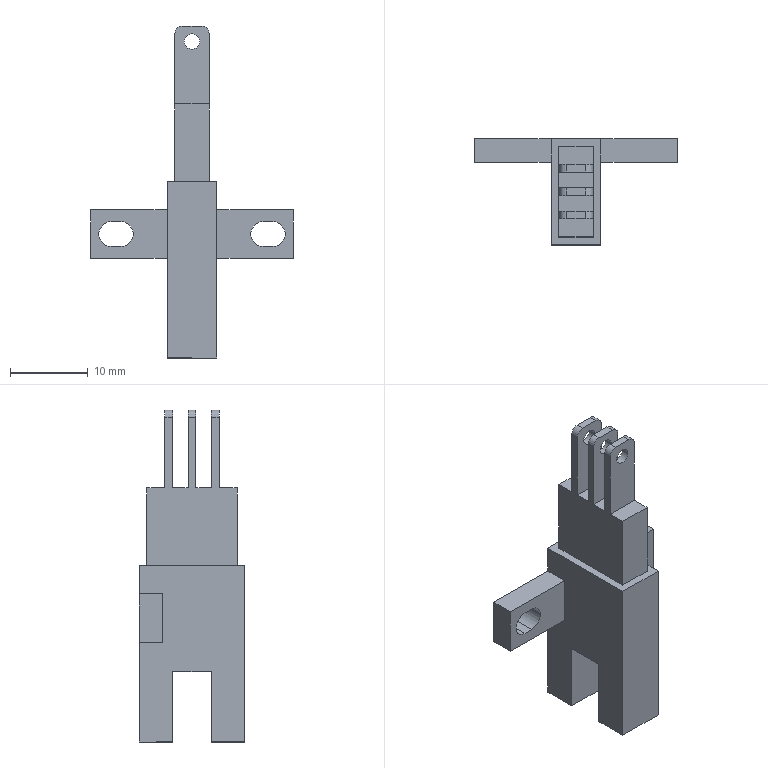Component | SolidWorks | U-shapedSensor-1 | 1 solid | 55 faces | box 26 x 13.6 x 42.6 mm | volume 2610 mm3 | plane 39 | cylinder 16 | commonest cylinder face diameters 2 x12 3.2 x4
build123d program:
from build123d import *

# Parameters (mm, degrees)
SKETCH1_W              = 13.6
SKETCH1_H              = 22.6
BOSS_EXTRUDE1_DEPTH    = 6.4
SKETCH2_W              = 4.9
SKETCH2_H              = 9
CUT_EXTRUDE1_DEPTH     = 28.142
SKETCH3_W              = 13
SKETCH3_H              = 6.2
BOSS_EXTRUDE2_DEPTH    = 3
CUT_EXTRUDE2_DEPTH     = 31.954
SKETCH5_W              = 11.6
SKETCH5_H              = 4.4
BOSS_EXTRUDE3_DEPTH    = 10
SKETCH6_W              = 1
SKETCH6_H              = 4.4
BOSS_EXTRUDE4_DEPTH    = 10
FILLET1_R              = 1
SKETCH7_R              = 1
CUT_EXTRUDE3_DEPTH     = 10
LPATTERN1_COUNT        = 2
LPATTERN1_PITCH        = 3
LPATTERN1_COUNT_DIR2   = 2
LPATTERN1_PITCH_DIR2   = 3
FILLET1_OF_LPATTERN1_R = 1


with BuildPart() as part:
    # Sketch1 → Boss-Extrude1 (new body)
    with BuildSketch(Plane.XY):
        with Locations((6.8, -11.3)):
            Rectangle(SKETCH1_W, SKETCH1_H)
    extrude(amount=BOSS_EXTRUDE1_DEPTH)

    # Sketch2 → Cut-Extrude1 (cut, through all)
    with BuildSketch(Plane.XY.offset(6.4)):
        with Locations((6.8, -4.5)):
            Rectangle(SKETCH2_W, SKETCH2_H)
    extrude(amount=-CUT_EXTRUDE1_DEPTH, mode=Mode.SUBTRACT)

    # Sketch3 → Boss-Extrude2 (add)
    with BuildSketch(Plane.ZY):
        with Locations((9.7, -15.9)):
            Rectangle(SKETCH3_W, SKETCH3_H)
    boss_extrude2 = extrude(amount=-BOSS_EXTRUDE2_DEPTH)

    # Sketch4 → Cut-Extrude2 (cut, through all)
    with BuildSketch(Plane.ZY):
        with BuildLine():
            Line((12.35, -14.3), (13.55, -14.3))
            ThreePointArc((13.55, -14.3), (15.15, -15.9), (13.55, -17.5))
            Line((13.55, -17.5), (12.35, -17.5))
            ThreePointArc((12.35, -17.5), (10.75, -15.9), (12.35, -14.3))
        make_face()
    cut_extrude2 = extrude(amount=-CUT_EXTRUDE2_DEPTH, mode=Mode.SUBTRACT)

    # Mirror1: Boss-Extrude2, Cut-Extrude2 across plane
    add(boss_extrude2.mirror(Plane(origin=(0, 0, 3.2), x_dir=(1, 0, 0), z_dir=(0, 0, -1))))
    add(cut_extrude2.mirror(Plane(origin=(0, 0, 3.2), x_dir=(1, 0, 0), z_dir=(0, 0, -1))), mode=Mode.SUBTRACT)

    # Sketch5 → Boss-Extrude3 (add)
    with BuildSketch(Plane.XZ.offset(22.6)):
        with Locations((6.8, 3.2)):
            Rectangle(SKETCH5_W, SKETCH5_H)
    extrude(amount=BOSS_EXTRUDE3_DEPTH)

    # Sketch6 → Boss-Extrude4 (add)
    with BuildSketch(Plane.XZ.offset(32.6)):
        with Locations((6.8, 3.2)):
            Rectangle(SKETCH6_W, SKETCH6_H)
    boss_extrude4 = extrude(amount=BOSS_EXTRUDE4_DEPTH)

    # Fillet1
    fillet1_edges = [part.edges().sort_by_distance(p)[0] for p in [
        (6.8, -42.6, 1),
        (6.8, -42.6, 5.4),
    ]]
    fillet(fillet1_edges, radius=FILLET1_R)

    # Sketch7 → Cut-Extrude3 (cut)
    with BuildSketch(Plane.ZY.offset(-6.3)):
        with Locations((3.2, -40.6)):
            Circle(SKETCH7_R)
    cut_extrude3 = extrude(amount=-CUT_EXTRUDE3_DEPTH, mode=Mode.SUBTRACT)

    # LPattern1: Boss-Extrude4, Cut-Extrude3 2 × 2
    with Locations(*[Vector(1, 0, 0) * (i * LPATTERN1_PITCH) + Vector(-1, 0, 0) * (j * LPATTERN1_PITCH_DIR2) for i in range(LPATTERN1_COUNT) for j in range(LPATTERN1_COUNT_DIR2) if (i, j) != (0, 0)]):
        add(boss_extrude4)
        add(cut_extrude3, mode=Mode.SUBTRACT)

    # Fillet1 of LPattern1
    fillet1_of_lpattern1_edges = [part.edges().sort_by_distance(p)[0] for p in [
        (3.8, -42.6, 1),
        (3.8, -42.6, 5.4),
        (9.8, -42.6, 1),
        (9.8, -42.6, 5.4),
        (6.8, -42.6, 1),
        (6.8, -42.6, 5.4),
    ]]
    fillet(fillet1_of_lpattern1_edges, radius=FILLET1_OF_LPATTERN1_R)


solid = part.part

# Placed as in the assembly
solid = solid.moved(Location((-140.872, -19.055, -25.349), (-90, 90, 0)))